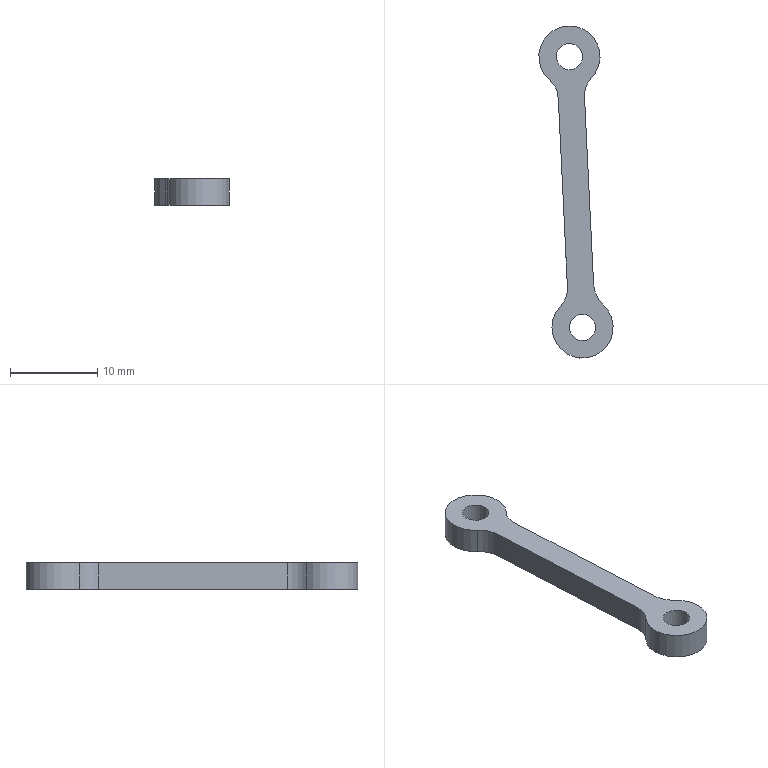Component | NX | LINK_2 | 1 solid | 12 faces | box 8.5 x 37.96 x 3 mm | volume 410 mm3 | cylinder 8 | plane 4 | commonest cylinder face diameters 6 x3 7 x2 3 x2 7.2 x1
STEP:
#1=CARTESIAN_POINT('',(0.,0.,0.));
#2=DIRECTION('',(0.,0.,1.));
#3=DIRECTION('',(1.,0.,0.));
#4=AXIS2_PLACEMENT_3D('',#1,#2,#3);
#5=CARTESIAN_POINT('',(7.782,-30.756,26.65));
#6=VERTEX_POINT('',#5);
#7=CARTESIAN_POINT('',(2.942,-30.99,26.65));
#8=VERTEX_POINT('',#7);
#9=CARTESIAN_POINT('',(5.24,-28.35,26.65));
#10=DIRECTION('',(0.,0.,1.));
#11=DIRECTION('',(0.04829,-0.9988,0.));
#12=AXIS2_PLACEMENT_3D('',#9,#10,#11);
#13=CIRCLE('',#12,3.5);
#14=CARTESIAN_POINT('',(5.24,-28.35,29.65));
#15=DIRECTION('',(0.,0.,-1.));
#16=DIRECTION('',(0.9988,0.04829,0.));
#17=AXIS2_PLACEMENT_3D('',#14,#15,#16);
#18=CYLINDRICAL_SURFACE('',#17,3.5);
#19=CARTESIAN_POINT('',(7.854,3.));
#20=DIRECTION('',(-1.,0.));
#21=VECTOR('',#20,1.);
#22=LINE('',#19,#21);
#23=(GEOMETRIC_REPRESENTATION_CONTEXT(2)PARAMETRIC_REPRESENTATION_CONTEXT()REPRESENTATION_CONTEXT('',''));
#24=DEFINITIONAL_REPRESENTATION('',(#22),#23);
#25=PCURVE('',#18,#24);
#26=CARTESIAN_POINT('',(5.24,-28.35,26.65));
#27=DIRECTION('',(0.,0.,1.));
#28=DIRECTION('',(-0.9988,-0.04829,0.));
#29=AXIS2_PLACEMENT_3D('',#26,#27,#28);
#30=PLANE('',#29);
#31=CARTESIAN_POINT('',(0.,0.));
#32=DIRECTION('',(0.,1.));
#33=AXIS2_PLACEMENT_2D('',#31,#32);
#34=CIRCLE('',#33,3.5);
#35=(GEOMETRIC_REPRESENTATION_CONTEXT(2)PARAMETRIC_REPRESENTATION_CONTEXT()REPRESENTATION_CONTEXT('',''));
#36=DEFINITIONAL_REPRESENTATION('',(#34),#35);
#37=PCURVE('',#30,#36);
#38=SURFACE_CURVE('',#13,(#25,#37),.PCURVE_S1.);
#39=EDGE_CURVE('',#6,#8,#38,.T.);
#40=ORIENTED_EDGE('',*,*,#39,.T.);
#41=CARTESIAN_POINT('',(2.942,-30.99,29.65));
#42=VERTEX_POINT('',#41);
#43=CARTESIAN_POINT('',(2.942,-30.99,29.65));
#44=DIRECTION('',(0.,0.,-1.));
#45=VECTOR('',#44,1.);
#46=LINE('',#43,#45);
#47=CARTESIAN_POINT('',(2.335,0.));
#48=DIRECTION('',(0.,1.));
#49=VECTOR('',#48,1.);
#50=LINE('',#47,#49);
#51=(GEOMETRIC_REPRESENTATION_CONTEXT(2)PARAMETRIC_REPRESENTATION_CONTEXT()REPRESENTATION_CONTEXT('',''));
#52=DEFINITIONAL_REPRESENTATION('',(#50),#51);
#53=PCURVE('',#18,#52);
#54=CARTESIAN_POINT('',(0.9717,-33.252,29.65));
#55=DIRECTION('',(0.,0.,-1.));
#56=DIRECTION('',(0.9988,0.04829,0.));
#57=AXIS2_PLACEMENT_3D('',#54,#55,#56);
#58=CYLINDRICAL_SURFACE('',#57,3.);
#59=CARTESIAN_POINT('',(5.477,0.));
#60=DIRECTION('',(0.,1.));
#61=VECTOR('',#60,1.);
#62=LINE('',#59,#61);
#63=(GEOMETRIC_REPRESENTATION_CONTEXT(2)PARAMETRIC_REPRESENTATION_CONTEXT()REPRESENTATION_CONTEXT('',''));
#64=DEFINITIONAL_REPRESENTATION('',(#62),#63);
#65=PCURVE('',#58,#64);
#66=SURFACE_CURVE('',#46,(#53,#65),.PCURVE_S1.);
#67=EDGE_CURVE('',#42,#8,#66,.T.);
#68=ORIENTED_EDGE('',*,*,#67,.F.);
#69=CARTESIAN_POINT('',(7.782,-30.756,29.65));
#70=VERTEX_POINT('',#69);
#71=CARTESIAN_POINT('',(5.24,-28.35,29.65));
#72=DIRECTION('',(0.,0.,1.));
#73=DIRECTION('',(0.04829,-0.9988,0.));
#74=AXIS2_PLACEMENT_3D('',#71,#72,#73);
#75=CIRCLE('',#74,3.5);
#76=CARTESIAN_POINT('',(7.854,0.));
#77=DIRECTION('',(-1.,0.));
#78=VECTOR('',#77,1.);
#79=LINE('',#76,#78);
#80=(GEOMETRIC_REPRESENTATION_CONTEXT(2)PARAMETRIC_REPRESENTATION_CONTEXT()REPRESENTATION_CONTEXT('',''));
#81=DEFINITIONAL_REPRESENTATION('',(#79),#80);
#82=PCURVE('',#18,#81);
#83=CARTESIAN_POINT('',(5.24,-28.35,29.65));
#84=DIRECTION('',(0.,0.,1.));
#85=DIRECTION('',(-0.9988,-0.04829,0.));
#86=AXIS2_PLACEMENT_3D('',#83,#84,#85);
#87=PLANE('',#86);
#88=CARTESIAN_POINT('',(0.,0.));
#89=DIRECTION('',(0.,1.));
#90=AXIS2_PLACEMENT_2D('',#88,#89);
#91=CIRCLE('',#90,3.5);
#92=(GEOMETRIC_REPRESENTATION_CONTEXT(2)PARAMETRIC_REPRESENTATION_CONTEXT()REPRESENTATION_CONTEXT('',''));
#93=DEFINITIONAL_REPRESENTATION('',(#91),#92);
#94=PCURVE('',#87,#93);
#95=SURFACE_CURVE('',#75,(#82,#94),.PCURVE_S1.);
#96=EDGE_CURVE('',#70,#42,#95,.T.);
#97=ORIENTED_EDGE('',*,*,#96,.F.);
#98=CARTESIAN_POINT('',(7.782,-30.756,29.65));
#99=DIRECTION('',(0.,0.,-1.));
#100=VECTOR('',#99,1.);
#101=LINE('',#98,#100);
#102=CARTESIAN_POINT('',(7.089,0.));
#103=DIRECTION('',(0.,1.));
#104=VECTOR('',#103,1.);
#105=LINE('',#102,#104);
#106=(GEOMETRIC_REPRESENTATION_CONTEXT(2)PARAMETRIC_REPRESENTATION_CONTEXT()REPRESENTATION_CONTEXT('',''));
#107=DEFINITIONAL_REPRESENTATION('',(#105),#106);
#108=PCURVE('',#18,#107);
#109=CARTESIAN_POINT('',(9.961,-32.818,29.65));
#110=DIRECTION('',(0.,0.,-1.));
#111=DIRECTION('',(0.9988,0.04829,0.));
#112=AXIS2_PLACEMENT_3D('',#109,#110,#111);
#113=CYLINDRICAL_SURFACE('',#112,3.);
#114=CARTESIAN_POINT('',(3.948,0.));
#115=DIRECTION('',(0.,1.));
#116=VECTOR('',#115,1.);
#117=LINE('',#114,#116);
#118=(GEOMETRIC_REPRESENTATION_CONTEXT(2)PARAMETRIC_REPRESENTATION_CONTEXT()REPRESENTATION_CONTEXT('',''));
#119=DEFINITIONAL_REPRESENTATION('',(#117),#118);
#120=PCURVE('',#113,#119);
#121=SURFACE_CURVE('',#101,(#108,#120),.PCURVE_S1.);
#122=EDGE_CURVE('',#70,#6,#121,.T.);
#123=ORIENTED_EDGE('',*,*,#122,.T.);
#124=EDGE_LOOP('',(#40,#68,#97,#123));
#125=FACE_BOUND('',#124,.T.);
#126=ADVANCED_FACE('',(#125),#18,.T.);
#127=ORIENTED_EDGE('',*,*,#67,.F.);
#128=CARTESIAN_POINT('',(3.968,-33.107,29.65));
#129=VERTEX_POINT('',#128);
#130=CARTESIAN_POINT('',(0.9717,-33.252,29.65));
#131=DIRECTION('',(0.,0.,-1.));
#132=DIRECTION('',(0.04829,-0.9988,0.));
#133=AXIS2_PLACEMENT_3D('',#130,#131,#132);
#134=CIRCLE('',#133,3.);
#135=CARTESIAN_POINT('',(1.571,0.));
#136=DIRECTION('',(1.,0.));
#137=VECTOR('',#136,1.);
#138=LINE('',#135,#137);
#139=(GEOMETRIC_REPRESENTATION_CONTEXT(2)PARAMETRIC_REPRESENTATION_CONTEXT()REPRESENTATION_CONTEXT('',''));
#140=DEFINITIONAL_REPRESENTATION('',(#138),#139);
#141=PCURVE('',#58,#140);
#142=CARTESIAN_POINT('',(4.5,7.69));
#143=CARTESIAN_POINT('',(9.696,7.69));
#144=CARTESIAN_POINT('',(7.098,3.19));
#145=CARTESIAN_POINT('',(4.5,-1.31));
#146=CARTESIAN_POINT('',(1.902,3.19));
#147=CARTESIAN_POINT('',(-0.6962,7.69));
#148=CARTESIAN_POINT('',(4.5,7.69));
#149=(BOUNDED_CURVE()B_SPLINE_CURVE(2,(#142,#143,#144,#145,#146,#147,#148),.UNSPECIFIED.,.T.,.F.)B_SPLINE_CURVE_WITH_KNOTS((1,2,2,2,2,1),(-2.094,0.,2.094,4.189,6.283,8.378),.UNSPECIFIED.)CURVE()GEOMETRIC_REPRESENTATION_ITEM()RATIONAL_B_SPLINE_CURVE((1.,0.5,1.,0.5,1.,0.5,1.))REPRESENTATION_ITEM(''));
#150=(GEOMETRIC_REPRESENTATION_CONTEXT(2)PARAMETRIC_REPRESENTATION_CONTEXT()REPRESENTATION_CONTEXT('',''));
#151=DEFINITIONAL_REPRESENTATION('',(#149),#150);
#152=PCURVE('',#87,#151);
#153=SURFACE_CURVE('',#134,(#141,#152),.PCURVE_S1.);
#154=EDGE_CURVE('',#42,#129,#153,.T.);
#155=ORIENTED_EDGE('',*,*,#154,.T.);
#156=CARTESIAN_POINT('',(3.968,-33.107,26.65));
#157=VERTEX_POINT('',#156);
#158=CARTESIAN_POINT('',(3.968,-33.107,29.65));
#159=DIRECTION('',(0.,0.,-1.));
#160=VECTOR('',#159,1.);
#161=LINE('',#158,#160);
#162=CARTESIAN_POINT('',(6.283,0.));
#163=DIRECTION('',(0.,1.));
#164=VECTOR('',#163,1.);
#165=LINE('',#162,#164);
#166=(GEOMETRIC_REPRESENTATION_CONTEXT(2)PARAMETRIC_REPRESENTATION_CONTEXT()REPRESENTATION_CONTEXT('',''));
#167=DEFINITIONAL_REPRESENTATION('',(#165),#166);
#168=PCURVE('',#58,#167);
#169=CARTESIAN_POINT('',(3.968,-33.107,29.65));
#170=DIRECTION('',(0.9988,0.04829,0.));
#171=DIRECTION('',(0.04829,-0.9988,0.));
#172=AXIS2_PLACEMENT_3D('',#169,#170,#171);
#173=PLANE('',#172);
#174=CARTESIAN_POINT('',(0.,0.));
#175=DIRECTION('',(0.,1.));
#176=VECTOR('',#175,1.);
#177=LINE('',#174,#176);
#178=(GEOMETRIC_REPRESENTATION_CONTEXT(2)PARAMETRIC_REPRESENTATION_CONTEXT()REPRESENTATION_CONTEXT('',''));
#179=DEFINITIONAL_REPRESENTATION('',(#177),#178);
#180=PCURVE('',#173,#179);
#181=SURFACE_CURVE('',#161,(#168,#180),.PCURVE_S1.);
#182=EDGE_CURVE('',#129,#157,#181,.T.);
#183=ORIENTED_EDGE('',*,*,#182,.T.);
#184=CARTESIAN_POINT('',(0.9717,-33.252,26.65));
#185=DIRECTION('',(0.,0.,-1.));
#186=DIRECTION('',(0.04829,-0.9988,0.));
#187=AXIS2_PLACEMENT_3D('',#184,#185,#186);
#188=CIRCLE('',#187,3.);
#189=CARTESIAN_POINT('',(1.571,3.));
#190=DIRECTION('',(1.,0.));
#191=VECTOR('',#190,1.);
#192=LINE('',#189,#191);
#193=(GEOMETRIC_REPRESENTATION_CONTEXT(2)PARAMETRIC_REPRESENTATION_CONTEXT()REPRESENTATION_CONTEXT('',''));
#194=DEFINITIONAL_REPRESENTATION('',(#192),#193);
#195=PCURVE('',#58,#194);
#196=CARTESIAN_POINT('',(4.5,7.69));
#197=CARTESIAN_POINT('',(9.696,7.69));
#198=CARTESIAN_POINT('',(7.098,3.19));
#199=CARTESIAN_POINT('',(4.5,-1.31));
#200=CARTESIAN_POINT('',(1.902,3.19));
#201=CARTESIAN_POINT('',(-0.6962,7.69));
#202=CARTESIAN_POINT('',(4.5,7.69));
#203=(BOUNDED_CURVE()B_SPLINE_CURVE(2,(#196,#197,#198,#199,#200,#201,#202),.UNSPECIFIED.,.T.,.F.)B_SPLINE_CURVE_WITH_KNOTS((1,2,2,2,2,1),(-2.094,0.,2.094,4.189,6.283,8.378),.UNSPECIFIED.)CURVE()GEOMETRIC_REPRESENTATION_ITEM()RATIONAL_B_SPLINE_CURVE((1.,0.5,1.,0.5,1.,0.5,1.))REPRESENTATION_ITEM(''));
#204=(GEOMETRIC_REPRESENTATION_CONTEXT(2)PARAMETRIC_REPRESENTATION_CONTEXT()REPRESENTATION_CONTEXT('',''));
#205=DEFINITIONAL_REPRESENTATION('',(#203),#204);
#206=PCURVE('',#30,#205);
#207=SURFACE_CURVE('',#188,(#195,#206),.PCURVE_S1.);
#208=EDGE_CURVE('',#8,#157,#207,.T.);
#209=ORIENTED_EDGE('',*,*,#208,.F.);
#210=EDGE_LOOP('',(#127,#155,#183,#209));
#211=FACE_BOUND('',#210,.F.);
#212=ADVANCED_FACE('',(#211),#58,.F.);
#213=CARTESIAN_POINT('',(5.012,-54.701,26.65));
#214=VERTEX_POINT('',#213);
#215=CARTESIAN_POINT('',(3.968,-33.107,26.65));
#216=DIRECTION('',(0.04829,-0.9988,0.));
#217=VECTOR('',#216,1.);
#218=LINE('',#215,#217);
#219=CARTESIAN_POINT('',(0.,3.));
#220=DIRECTION('',(1.,0.));
#221=VECTOR('',#220,1.);
#222=LINE('',#219,#221);
#223=(GEOMETRIC_REPRESENTATION_CONTEXT(2)PARAMETRIC_REPRESENTATION_CONTEXT()REPRESENTATION_CONTEXT('',''));
#224=DEFINITIONAL_REPRESENTATION('',(#222),#223);
#225=PCURVE('',#173,#224);
#226=CARTESIAN_POINT('',(1.5,4.69));
#227=DIRECTION('',(0.,1.));
#228=VECTOR('',#227,1.);
#229=LINE('',#226,#228);
#230=(GEOMETRIC_REPRESENTATION_CONTEXT(2)PARAMETRIC_REPRESENTATION_CONTEXT()REPRESENTATION_CONTEXT('',''));
#231=DEFINITIONAL_REPRESENTATION('',(#229),#230);
#232=PCURVE('',#30,#231);
#233=SURFACE_CURVE('',#218,(#225,#232),.PCURVE_S1.);
#234=EDGE_CURVE('',#157,#214,#233,.T.);
#235=ORIENTED_EDGE('',*,*,#234,.T.);
#236=CARTESIAN_POINT('',(5.012,-54.701,29.65));
#237=VERTEX_POINT('',#236);
#238=CARTESIAN_POINT('',(5.012,-54.701,29.65));
#239=DIRECTION('',(0.,0.,-1.));
#240=VECTOR('',#239,1.);
#241=LINE('',#238,#240);
#242=CARTESIAN_POINT('',(21.619,0.));
#243=DIRECTION('',(0.,1.));
#244=VECTOR('',#243,1.);
#245=LINE('',#242,#244);
#246=(GEOMETRIC_REPRESENTATION_CONTEXT(2)PARAMETRIC_REPRESENTATION_CONTEXT()REPRESENTATION_CONTEXT('',''));
#247=DEFINITIONAL_REPRESENTATION('',(#245),#246);
#248=PCURVE('',#173,#247);
#249=CARTESIAN_POINT('',(2.016,-54.846,29.65));
#250=DIRECTION('',(0.,0.,-1.));
#251=DIRECTION('',(0.9988,0.04829,0.));
#252=AXIS2_PLACEMENT_3D('',#249,#250,#251);
#253=CYLINDRICAL_SURFACE('',#252,3.);
#254=CARTESIAN_POINT('',(0.,0.));
#255=DIRECTION('',(0.,1.));
#256=VECTOR('',#255,1.);
#257=LINE('',#254,#256);
#258=(GEOMETRIC_REPRESENTATION_CONTEXT(2)PARAMETRIC_REPRESENTATION_CONTEXT()REPRESENTATION_CONTEXT('',''));
#259=DEFINITIONAL_REPRESENTATION('',(#257),#258);
#260=PCURVE('',#253,#259);
#261=SURFACE_CURVE('',#241,(#248,#260),.PCURVE_S1.);
#262=EDGE_CURVE('',#237,#214,#261,.T.);
#263=ORIENTED_EDGE('',*,*,#262,.F.);
#264=CARTESIAN_POINT('',(3.968,-33.107,29.65));
#265=DIRECTION('',(0.04829,-0.9988,0.));
#266=VECTOR('',#265,1.);
#267=LINE('',#264,#266);
#268=CARTESIAN_POINT('',(0.,0.));
#269=DIRECTION('',(1.,0.));
#270=VECTOR('',#269,1.);
#271=LINE('',#268,#270);
#272=(GEOMETRIC_REPRESENTATION_CONTEXT(2)PARAMETRIC_REPRESENTATION_CONTEXT()REPRESENTATION_CONTEXT('',''));
#273=DEFINITIONAL_REPRESENTATION('',(#271),#272);
#274=PCURVE('',#173,#273);
#275=CARTESIAN_POINT('',(1.5,4.69));
#276=DIRECTION('',(0.,1.));
#277=VECTOR('',#276,1.);
#278=LINE('',#275,#277);
#279=(GEOMETRIC_REPRESENTATION_CONTEXT(2)PARAMETRIC_REPRESENTATION_CONTEXT()REPRESENTATION_CONTEXT('',''));
#280=DEFINITIONAL_REPRESENTATION('',(#278),#279);
#281=PCURVE('',#87,#280);
#282=SURFACE_CURVE('',#267,(#274,#281),.PCURVE_S1.);
#283=EDGE_CURVE('',#129,#237,#282,.T.);
#284=ORIENTED_EDGE('',*,*,#283,.F.);
#285=ORIENTED_EDGE('',*,*,#182,.T.);
#286=EDGE_LOOP('',(#235,#263,#284,#285));
#287=FACE_BOUND('',#286,.T.);
#288=ADVANCED_FACE('',(#287),#173,.F.);
#289=ORIENTED_EDGE('',*,*,#262,.F.);
#290=CARTESIAN_POINT('',(4.195,-56.908,29.65));
#291=VERTEX_POINT('',#290);
#292=CARTESIAN_POINT('',(2.016,-54.846,29.65));
#293=DIRECTION('',(0.,0.,-1.));
#294=DIRECTION('',(0.04829,-0.9988,0.));
#295=AXIS2_PLACEMENT_3D('',#292,#293,#294);
#296=CIRCLE('',#295,3.);
#297=CARTESIAN_POINT('',(-4.712,0.));
#298=DIRECTION('',(1.,0.));
#299=VECTOR('',#298,1.);
#300=LINE('',#297,#299);
#301=(GEOMETRIC_REPRESENTATION_CONTEXT(2)PARAMETRIC_REPRESENTATION_CONTEXT()REPRESENTATION_CONTEXT('',''));
#302=DEFINITIONAL_REPRESENTATION('',(#300),#301);
#303=PCURVE('',#253,#302);
#304=CARTESIAN_POINT('',(4.5,29.31));
#305=CARTESIAN_POINT('',(9.696,29.31));
#306=CARTESIAN_POINT('',(7.098,24.81));
#307=CARTESIAN_POINT('',(4.5,20.31));
#308=CARTESIAN_POINT('',(1.902,24.81));
#309=CARTESIAN_POINT('',(-0.6962,29.31));
#310=CARTESIAN_POINT('',(4.5,29.31));
#311=(BOUNDED_CURVE()B_SPLINE_CURVE(2,(#304,#305,#306,#307,#308,#309,#310),.UNSPECIFIED.,.T.,.F.)B_SPLINE_CURVE_WITH_KNOTS((1,2,2,2,2,1),(-2.094,0.,2.094,4.189,6.283,8.378),.UNSPECIFIED.)CURVE()GEOMETRIC_REPRESENTATION_ITEM()RATIONAL_B_SPLINE_CURVE((1.,0.5,1.,0.5,1.,0.5,1.))REPRESENTATION_ITEM(''));
#312=(GEOMETRIC_REPRESENTATION_CONTEXT(2)PARAMETRIC_REPRESENTATION_CONTEXT()REPRESENTATION_CONTEXT('',''));
#313=DEFINITIONAL_REPRESENTATION('',(#311),#312);
#314=PCURVE('',#87,#313);
#315=SURFACE_CURVE('',#296,(#303,#314),.PCURVE_S1.);
#316=EDGE_CURVE('',#237,#291,#315,.T.);
#317=ORIENTED_EDGE('',*,*,#316,.T.);
#318=CARTESIAN_POINT('',(4.195,-56.908,26.65));
#319=VERTEX_POINT('',#318);
#320=CARTESIAN_POINT('',(4.195,-56.908,29.65));
#321=DIRECTION('',(0.,0.,-1.));
#322=VECTOR('',#321,1.);
#323=LINE('',#320,#322);
#324=CARTESIAN_POINT('',(0.8061,0.));
#325=DIRECTION('',(0.,1.));
#326=VECTOR('',#325,1.);
#327=LINE('',#324,#326);
#328=(GEOMETRIC_REPRESENTATION_CONTEXT(2)PARAMETRIC_REPRESENTATION_CONTEXT()REPRESENTATION_CONTEXT('',''));
#329=DEFINITIONAL_REPRESENTATION('',(#327),#328);
#330=PCURVE('',#253,#329);
#331=CARTESIAN_POINT('',(6.737,-59.314,29.65));
#332=DIRECTION('',(0.,0.,-1.));
#333=DIRECTION('',(0.9988,0.04829,0.));
#334=AXIS2_PLACEMENT_3D('',#331,#332,#333);
#335=CYLINDRICAL_SURFACE('',#334,3.5);
#336=CARTESIAN_POINT('',(3.948,0.));
#337=DIRECTION('',(0.,1.));
#338=VECTOR('',#337,1.);
#339=LINE('',#336,#338);
#340=(GEOMETRIC_REPRESENTATION_CONTEXT(2)PARAMETRIC_REPRESENTATION_CONTEXT()REPRESENTATION_CONTEXT('',''));
#341=DEFINITIONAL_REPRESENTATION('',(#339),#340);
#342=PCURVE('',#335,#341);
#343=SURFACE_CURVE('',#323,(#330,#342),.PCURVE_S1.);
#344=EDGE_CURVE('',#291,#319,#343,.T.);
#345=ORIENTED_EDGE('',*,*,#344,.T.);
#346=CARTESIAN_POINT('',(2.016,-54.846,26.65));
#347=DIRECTION('',(0.,0.,-1.));
#348=DIRECTION('',(0.04829,-0.9988,0.));
#349=AXIS2_PLACEMENT_3D('',#346,#347,#348);
#350=CIRCLE('',#349,3.);
#351=CARTESIAN_POINT('',(-4.712,3.));
#352=DIRECTION('',(1.,0.));
#353=VECTOR('',#352,1.);
#354=LINE('',#351,#353);
#355=(GEOMETRIC_REPRESENTATION_CONTEXT(2)PARAMETRIC_REPRESENTATION_CONTEXT()REPRESENTATION_CONTEXT('',''));
#356=DEFINITIONAL_REPRESENTATION('',(#354),#355);
#357=PCURVE('',#253,#356);
#358=CARTESIAN_POINT('',(4.5,29.31));
#359=CARTESIAN_POINT('',(9.696,29.31));
#360=CARTESIAN_POINT('',(7.098,24.81));
#361=CARTESIAN_POINT('',(4.5,20.31));
#362=CARTESIAN_POINT('',(1.902,24.81));
#363=CARTESIAN_POINT('',(-0.6962,29.31));
#364=CARTESIAN_POINT('',(4.5,29.31));
#365=(BOUNDED_CURVE()B_SPLINE_CURVE(2,(#358,#359,#360,#361,#362,#363,#364),.UNSPECIFIED.,.T.,.F.)B_SPLINE_CURVE_WITH_KNOTS((1,2,2,2,2,1),(-2.094,0.,2.094,4.189,6.283,8.378),.UNSPECIFIED.)CURVE()GEOMETRIC_REPRESENTATION_ITEM()RATIONAL_B_SPLINE_CURVE((1.,0.5,1.,0.5,1.,0.5,1.))REPRESENTATION_ITEM(''));
#366=(GEOMETRIC_REPRESENTATION_CONTEXT(2)PARAMETRIC_REPRESENTATION_CONTEXT()REPRESENTATION_CONTEXT('',''));
#367=DEFINITIONAL_REPRESENTATION('',(#365),#366);
#368=PCURVE('',#30,#367);
#369=SURFACE_CURVE('',#350,(#357,#368),.PCURVE_S1.);
#370=EDGE_CURVE('',#214,#319,#369,.T.);
#371=ORIENTED_EDGE('',*,*,#370,.F.);
#372=EDGE_LOOP('',(#289,#317,#345,#371));
#373=FACE_BOUND('',#372,.F.);
#374=ADVANCED_FACE('',(#373),#253,.F.);
#375=CARTESIAN_POINT('',(9.13,-56.76,26.65));
#376=VERTEX_POINT('',#375);
#377=CARTESIAN_POINT('',(6.737,-59.314,26.65));
#378=DIRECTION('',(0.,0.,1.));
#379=DIRECTION('',(0.04829,-0.9988,0.));
#380=AXIS2_PLACEMENT_3D('',#377,#378,#379);
#381=CIRCLE('',#380,3.5);
#382=CARTESIAN_POINT('',(7.854,3.));
#383=DIRECTION('',(-1.,0.));
#384=VECTOR('',#383,1.);
#385=LINE('',#382,#384);
#386=(GEOMETRIC_REPRESENTATION_CONTEXT(2)PARAMETRIC_REPRESENTATION_CONTEXT()REPRESENTATION_CONTEXT('',''));
#387=DEFINITIONAL_REPRESENTATION('',(#385),#386);
#388=PCURVE('',#335,#387);
#389=CARTESIAN_POINT('',(0.,31.));
#390=DIRECTION('',(0.,1.));
#391=AXIS2_PLACEMENT_2D('',#389,#390);
#392=CIRCLE('',#391,3.5);
#393=(GEOMETRIC_REPRESENTATION_CONTEXT(2)PARAMETRIC_REPRESENTATION_CONTEXT()REPRESENTATION_CONTEXT('',''));
#394=DEFINITIONAL_REPRESENTATION('',(#392),#393);
#395=PCURVE('',#30,#394);
#396=SURFACE_CURVE('',#381,(#388,#395),.PCURVE_S1.);
#397=EDGE_CURVE('',#319,#376,#396,.T.);
#398=ORIENTED_EDGE('',*,*,#397,.T.);
#399=CARTESIAN_POINT('',(9.13,-56.76,29.65));
#400=VERTEX_POINT('',#399);
#401=CARTESIAN_POINT('',(9.13,-56.76,29.65));
#402=DIRECTION('',(0.,0.,-1.));
#403=VECTOR('',#402,1.);
#404=LINE('',#401,#403);
#405=CARTESIAN_POINT('',(-0.7694,0.));
#406=DIRECTION('',(0.,1.));
#407=VECTOR('',#406,1.);
#408=LINE('',#405,#407);
#409=(GEOMETRIC_REPRESENTATION_CONTEXT(2)PARAMETRIC_REPRESENTATION_CONTEXT()REPRESENTATION_CONTEXT('',''));
#410=DEFINITIONAL_REPRESENTATION('',(#408),#409);
#411=PCURVE('',#335,#410);
#412=CARTESIAN_POINT('',(11.592,-54.134,29.65));
#413=DIRECTION('',(0.,0.,-1.));
#414=DIRECTION('',(0.9988,0.04829,0.));
#415=AXIS2_PLACEMENT_3D('',#412,#413,#414);
#416=CYLINDRICAL_SURFACE('',#415,3.6);
#417=CARTESIAN_POINT('',(2.372,0.));
#418=DIRECTION('',(0.,1.));
#419=VECTOR('',#418,1.);
#420=LINE('',#417,#419);
#421=(GEOMETRIC_REPRESENTATION_CONTEXT(2)PARAMETRIC_REPRESENTATION_CONTEXT()REPRESENTATION_CONTEXT('',''));
#422=DEFINITIONAL_REPRESENTATION('',(#420),#421);
#423=PCURVE('',#416,#422);
#424=SURFACE_CURVE('',#404,(#411,#423),.PCURVE_S1.);
#425=EDGE_CURVE('',#400,#376,#424,.T.);
#426=ORIENTED_EDGE('',*,*,#425,.F.);
#427=CARTESIAN_POINT('',(6.737,-59.314,29.65));
#428=DIRECTION('',(0.,0.,1.));
#429=DIRECTION('',(0.04829,-0.9988,0.));
#430=AXIS2_PLACEMENT_3D('',#427,#428,#429);
#431=CIRCLE('',#430,3.5);
#432=CARTESIAN_POINT('',(7.854,0.));
#433=DIRECTION('',(-1.,0.));
#434=VECTOR('',#433,1.);
#435=LINE('',#432,#434);
#436=(GEOMETRIC_REPRESENTATION_CONTEXT(2)PARAMETRIC_REPRESENTATION_CONTEXT()REPRESENTATION_CONTEXT('',''));
#437=DEFINITIONAL_REPRESENTATION('',(#435),#436);
#438=PCURVE('',#335,#437);
#439=CARTESIAN_POINT('',(0.,31.));
#440=DIRECTION('',(0.,1.));
#441=AXIS2_PLACEMENT_2D('',#439,#440);
#442=CIRCLE('',#441,3.5);
#443=(GEOMETRIC_REPRESENTATION_CONTEXT(2)PARAMETRIC_REPRESENTATION_CONTEXT()REPRESENTATION_CONTEXT('',''));
#444=DEFINITIONAL_REPRESENTATION('',(#442),#443);
#445=PCURVE('',#87,#444);
#446=SURFACE_CURVE('',#431,(#438,#445),.PCURVE_S1.);
#447=EDGE_CURVE('',#291,#400,#446,.T.);
#448=ORIENTED_EDGE('',*,*,#447,.F.);
#449=ORIENTED_EDGE('',*,*,#344,.T.);
#450=EDGE_LOOP('',(#398,#426,#448,#449));
#451=FACE_BOUND('',#450,.T.);
#452=ADVANCED_FACE('',(#451),#335,.T.);
#453=ORIENTED_EDGE('',*,*,#425,.F.);
#454=CARTESIAN_POINT('',(7.997,-54.308,29.65));
#455=VERTEX_POINT('',#454);
#456=CARTESIAN_POINT('',(11.592,-54.134,29.65));
#457=DIRECTION('',(0.,0.,-1.));
#458=DIRECTION('',(0.04829,-0.9988,0.));
#459=AXIS2_PLACEMENT_3D('',#456,#457,#458);
#460=CIRCLE('',#459,3.6);
#461=CARTESIAN_POINT('',(1.571,0.));
#462=DIRECTION('',(1.,0.));
#463=VECTOR('',#462,1.);
#464=LINE('',#461,#463);
#465=(GEOMETRIC_REPRESENTATION_CONTEXT(2)PARAMETRIC_REPRESENTATION_CONTEXT()REPRESENTATION_CONTEXT('',''));
#466=DEFINITIONAL_REPRESENTATION('',(#464),#465);
#467=PCURVE('',#416,#466);
#468=CARTESIAN_POINT('',(-5.1,29.66));
#469=CARTESIAN_POINT('',(1.135,29.66));
#470=CARTESIAN_POINT('',(-1.982,24.26));
#471=CARTESIAN_POINT('',(-5.1,18.86));
#472=CARTESIAN_POINT('',(-8.218,24.26));
#473=CARTESIAN_POINT('',(-11.335,29.66));
#474=CARTESIAN_POINT('',(-5.1,29.66));
#475=(BOUNDED_CURVE()B_SPLINE_CURVE(2,(#468,#469,#470,#471,#472,#473,#474),.UNSPECIFIED.,.T.,.F.)B_SPLINE_CURVE_WITH_KNOTS((1,2,2,2,2,1),(-2.094,0.,2.094,4.189,6.283,8.378),.UNSPECIFIED.)CURVE()GEOMETRIC_REPRESENTATION_ITEM()RATIONAL_B_SPLINE_CURVE((1.,0.5,1.,0.5,1.,0.5,1.))REPRESENTATION_ITEM(''));
#476=(GEOMETRIC_REPRESENTATION_CONTEXT(2)PARAMETRIC_REPRESENTATION_CONTEXT()REPRESENTATION_CONTEXT('',''));
#477=DEFINITIONAL_REPRESENTATION('',(#475),#476);
#478=PCURVE('',#87,#477);
#479=SURFACE_CURVE('',#460,(#467,#478),.PCURVE_S1.);
#480=EDGE_CURVE('',#400,#455,#479,.T.);
#481=ORIENTED_EDGE('',*,*,#480,.T.);
#482=CARTESIAN_POINT('',(7.997,-54.308,26.65));
#483=VERTEX_POINT('',#482);
#484=CARTESIAN_POINT('',(7.997,-54.308,29.65));
#485=DIRECTION('',(0.,0.,-1.));
#486=VECTOR('',#485,1.);
#487=LINE('',#484,#486);
#488=CARTESIAN_POINT('',(3.142,0.));
#489=DIRECTION('',(0.,1.));
#490=VECTOR('',#489,1.);
#491=LINE('',#488,#490);
#492=(GEOMETRIC_REPRESENTATION_CONTEXT(2)PARAMETRIC_REPRESENTATION_CONTEXT()REPRESENTATION_CONTEXT('',''));
#493=DEFINITIONAL_REPRESENTATION('',(#491),#492);
#494=PCURVE('',#416,#493);
#495=CARTESIAN_POINT('',(7.997,-54.308,29.65));
#496=DIRECTION('',(-0.9988,-0.04829,0.));
#497=DIRECTION('',(-0.04829,0.9988,0.));
#498=AXIS2_PLACEMENT_3D('',#495,#496,#497);
#499=PLANE('',#498);
#500=CARTESIAN_POINT('',(0.,0.));
#501=DIRECTION('',(0.,1.));
#502=VECTOR('',#501,1.);
#503=LINE('',#500,#502);
#504=(GEOMETRIC_REPRESENTATION_CONTEXT(2)PARAMETRIC_REPRESENTATION_CONTEXT()REPRESENTATION_CONTEXT('',''));
#505=DEFINITIONAL_REPRESENTATION('',(#503),#504);
#506=PCURVE('',#499,#505);
#507=SURFACE_CURVE('',#487,(#494,#506),.PCURVE_S1.);
#508=EDGE_CURVE('',#455,#483,#507,.T.);
#509=ORIENTED_EDGE('',*,*,#508,.T.);
#510=CARTESIAN_POINT('',(11.592,-54.134,26.65));
#511=DIRECTION('',(0.,0.,-1.));
#512=DIRECTION('',(0.04829,-0.9988,0.));
#513=AXIS2_PLACEMENT_3D('',#510,#511,#512);
#514=CIRCLE('',#513,3.6);
#515=CARTESIAN_POINT('',(1.571,3.));
#516=DIRECTION('',(1.,0.));
#517=VECTOR('',#516,1.);
#518=LINE('',#515,#517);
#519=(GEOMETRIC_REPRESENTATION_CONTEXT(2)PARAMETRIC_REPRESENTATION_CONTEXT()REPRESENTATION_CONTEXT('',''));
#520=DEFINITIONAL_REPRESENTATION('',(#518),#519);
#521=PCURVE('',#416,#520);
#522=CARTESIAN_POINT('',(-5.1,29.66));
#523=CARTESIAN_POINT('',(1.135,29.66));
#524=CARTESIAN_POINT('',(-1.982,24.26));
#525=CARTESIAN_POINT('',(-5.1,18.86));
#526=CARTESIAN_POINT('',(-8.218,24.26));
#527=CARTESIAN_POINT('',(-11.335,29.66));
#528=CARTESIAN_POINT('',(-5.1,29.66));
#529=(BOUNDED_CURVE()B_SPLINE_CURVE(2,(#522,#523,#524,#525,#526,#527,#528),.UNSPECIFIED.,.T.,.F.)B_SPLINE_CURVE_WITH_KNOTS((1,2,2,2,2,1),(-2.094,0.,2.094,4.189,6.283,8.378),.UNSPECIFIED.)CURVE()GEOMETRIC_REPRESENTATION_ITEM()RATIONAL_B_SPLINE_CURVE((1.,0.5,1.,0.5,1.,0.5,1.))REPRESENTATION_ITEM(''));
#530=(GEOMETRIC_REPRESENTATION_CONTEXT(2)PARAMETRIC_REPRESENTATION_CONTEXT()REPRESENTATION_CONTEXT('',''));
#531=DEFINITIONAL_REPRESENTATION('',(#529),#530);
#532=PCURVE('',#30,#531);
#533=SURFACE_CURVE('',#514,(#521,#532),.PCURVE_S1.);
#534=EDGE_CURVE('',#376,#483,#533,.T.);
#535=ORIENTED_EDGE('',*,*,#534,.F.);
#536=EDGE_LOOP('',(#453,#481,#509,#535));
#537=FACE_BOUND('',#536,.F.);
#538=ADVANCED_FACE('',(#537),#416,.F.);
#539=CARTESIAN_POINT('',(6.965,-32.963,26.65));
#540=VERTEX_POINT('',#539);
#541=CARTESIAN_POINT('',(7.997,-54.308,26.65));
#542=DIRECTION('',(-0.04829,0.9988,0.));
#543=VECTOR('',#542,1.);
#544=LINE('',#541,#543);
#545=CARTESIAN_POINT('',(0.,3.));
#546=DIRECTION('',(1.,0.));
#547=VECTOR('',#546,1.);
#548=LINE('',#545,#547);
#549=(GEOMETRIC_REPRESENTATION_CONTEXT(2)PARAMETRIC_REPRESENTATION_CONTEXT()REPRESENTATION_CONTEXT('',''));
#550=DEFINITIONAL_REPRESENTATION('',(#548),#549);
#551=PCURVE('',#499,#550);
#552=CARTESIAN_POINT('',(-1.5,26.06));
#553=DIRECTION('',(0.,-1.));
#554=VECTOR('',#553,1.);
#555=LINE('',#552,#554);
#556=(GEOMETRIC_REPRESENTATION_CONTEXT(2)PARAMETRIC_REPRESENTATION_CONTEXT()REPRESENTATION_CONTEXT('',''));
#557=DEFINITIONAL_REPRESENTATION('',(#555),#556);
#558=PCURVE('',#30,#557);
#559=SURFACE_CURVE('',#544,(#551,#558),.PCURVE_S1.);
#560=EDGE_CURVE('',#483,#540,#559,.T.);
#561=ORIENTED_EDGE('',*,*,#560,.T.);
#562=CARTESIAN_POINT('',(6.965,-32.963,29.65));
#563=VERTEX_POINT('',#562);
#564=CARTESIAN_POINT('',(6.965,-32.963,29.65));
#565=DIRECTION('',(0.,0.,-1.));
#566=VECTOR('',#565,1.);
#567=LINE('',#564,#566);
#568=CARTESIAN_POINT('',(21.37,0.));
#569=DIRECTION('',(0.,1.));
#570=VECTOR('',#569,1.);
#571=LINE('',#568,#570);
#572=(GEOMETRIC_REPRESENTATION_CONTEXT(2)PARAMETRIC_REPRESENTATION_CONTEXT()REPRESENTATION_CONTEXT('',''));
#573=DEFINITIONAL_REPRESENTATION('',(#571),#572);
#574=PCURVE('',#499,#573);
#575=CARTESIAN_POINT('',(3.142,0.));
#576=DIRECTION('',(0.,1.));
#577=VECTOR('',#576,1.);
#578=LINE('',#575,#577);
#579=(GEOMETRIC_REPRESENTATION_CONTEXT(2)PARAMETRIC_REPRESENTATION_CONTEXT()REPRESENTATION_CONTEXT('',''));
#580=DEFINITIONAL_REPRESENTATION('',(#578),#579);
#581=PCURVE('',#113,#580);
#582=SURFACE_CURVE('',#567,(#574,#581),.PCURVE_S1.);
#583=EDGE_CURVE('',#563,#540,#582,.T.);
#584=ORIENTED_EDGE('',*,*,#583,.F.);
#585=CARTESIAN_POINT('',(7.997,-54.308,29.65));
#586=DIRECTION('',(-0.04829,0.9988,0.));
#587=VECTOR('',#586,1.);
#588=LINE('',#585,#587);
#589=CARTESIAN_POINT('',(0.,0.));
#590=DIRECTION('',(1.,0.));
#591=VECTOR('',#590,1.);
#592=LINE('',#589,#591);
#593=(GEOMETRIC_REPRESENTATION_CONTEXT(2)PARAMETRIC_REPRESENTATION_CONTEXT()REPRESENTATION_CONTEXT('',''));
#594=DEFINITIONAL_REPRESENTATION('',(#592),#593);
#595=PCURVE('',#499,#594);
#596=CARTESIAN_POINT('',(-1.5,26.06));
#597=DIRECTION('',(0.,-1.));
#598=VECTOR('',#597,1.);
#599=LINE('',#596,#598);
#600=(GEOMETRIC_REPRESENTATION_CONTEXT(2)PARAMETRIC_REPRESENTATION_CONTEXT()REPRESENTATION_CONTEXT('',''));
#601=DEFINITIONAL_REPRESENTATION('',(#599),#600);
#602=PCURVE('',#87,#601);
#603=SURFACE_CURVE('',#588,(#595,#602),.PCURVE_S1.);
#604=EDGE_CURVE('',#455,#563,#603,.T.);
#605=ORIENTED_EDGE('',*,*,#604,.F.);
#606=ORIENTED_EDGE('',*,*,#508,.T.);
#607=EDGE_LOOP('',(#561,#584,#605,#606));
#608=FACE_BOUND('',#607,.T.);
#609=ADVANCED_FACE('',(#608),#499,.F.);
#610=CARTESIAN_POINT('',(5.312,-29.848,29.65));
#611=VERTEX_POINT('',#610);
#612=CARTESIAN_POINT('',(5.24,-28.35,29.65));
#613=DIRECTION('',(0.,0.,1.));
#614=DIRECTION('',(0.04829,-0.9988,0.));
#615=AXIS2_PLACEMENT_3D('',#612,#613,#614);
#616=CIRCLE('',#615,1.5);
#617=CARTESIAN_POINT('',(5.24,-28.35,29.65));
#618=DIRECTION('',(0.,0.,-1.));
#619=DIRECTION('',(0.9988,0.04829,0.));
#620=AXIS2_PLACEMENT_3D('',#617,#618,#619);
#621=CYLINDRICAL_SURFACE('',#620,1.5);
#622=CARTESIAN_POINT('',(7.854,0.));
#623=DIRECTION('',(-1.,0.));
#624=VECTOR('',#623,1.);
#625=LINE('',#622,#624);
#626=(GEOMETRIC_REPRESENTATION_CONTEXT(2)PARAMETRIC_REPRESENTATION_CONTEXT()REPRESENTATION_CONTEXT('',''));
#627=DEFINITIONAL_REPRESENTATION('',(#625),#626);
#628=PCURVE('',#621,#627);
#629=CARTESIAN_POINT('',(0.,0.));
#630=DIRECTION('',(0.,1.));
#631=AXIS2_PLACEMENT_2D('',#629,#630);
#632=CIRCLE('',#631,1.5);
#633=(GEOMETRIC_REPRESENTATION_CONTEXT(2)PARAMETRIC_REPRESENTATION_CONTEXT()REPRESENTATION_CONTEXT('',''));
#634=DEFINITIONAL_REPRESENTATION('',(#632),#633);
#635=PCURVE('',#87,#634);
#636=SURFACE_CURVE('',#616,(#628,#635),.PCURVE_S1.);
#637=EDGE_CURVE('',#611,#611,#636,.T.);
#638=ORIENTED_EDGE('',*,*,#637,.F.);
#639=CARTESIAN_POINT('',(5.312,-29.848,26.65));
#640=VERTEX_POINT('',#639);
#641=CARTESIAN_POINT('',(5.312,-29.848,29.65));
#642=CARTESIAN_POINT('',(5.312,-29.848,26.65));
#643=B_SPLINE_CURVE_WITH_KNOTS('',1,(#641,#642),.UNSPECIFIED.,.F.,.F.,(2,2),(0.,3.),.PIECEWISE_BEZIER_KNOTS.);
#644=CARTESIAN_POINT('',(7.854,0.));
#645=DIRECTION('',(0.,1.));
#646=VECTOR('',#645,1.);
#647=LINE('',#644,#646);
#648=(GEOMETRIC_REPRESENTATION_CONTEXT(2)PARAMETRIC_REPRESENTATION_CONTEXT()REPRESENTATION_CONTEXT('',''));
#649=DEFINITIONAL_REPRESENTATION('',(#647),#648);
#650=PCURVE('',#621,#649);
#651=CARTESIAN_POINT('',(1.571,0.));
#652=DIRECTION('',(0.,1.));
#653=VECTOR('',#652,1.);
#654=LINE('',#651,#653);
#655=(GEOMETRIC_REPRESENTATION_CONTEXT(2)PARAMETRIC_REPRESENTATION_CONTEXT()REPRESENTATION_CONTEXT('',''));
#656=DEFINITIONAL_REPRESENTATION('',(#654),#655);
#657=PCURVE('',#621,#656);
#658=SEAM_CURVE('',#643,(#650,#657),.PCURVE_S1.);
#659=EDGE_CURVE('',#611,#640,#658,.T.);
#660=ORIENTED_EDGE('',*,*,#659,.T.);
#661=CARTESIAN_POINT('',(5.24,-28.35,26.65));
#662=DIRECTION('',(0.,0.,1.));
#663=DIRECTION('',(0.04829,-0.9988,0.));
#664=AXIS2_PLACEMENT_3D('',#661,#662,#663);
#665=CIRCLE('',#664,1.5);
#666=CARTESIAN_POINT('',(7.854,3.));
#667=DIRECTION('',(-1.,0.));
#668=VECTOR('',#667,1.);
#669=LINE('',#666,#668);
#670=(GEOMETRIC_REPRESENTATION_CONTEXT(2)PARAMETRIC_REPRESENTATION_CONTEXT()REPRESENTATION_CONTEXT('',''));
#671=DEFINITIONAL_REPRESENTATION('',(#669),#670);
#672=PCURVE('',#621,#671);
#673=CARTESIAN_POINT('',(0.,0.));
#674=DIRECTION('',(0.,1.));
#675=AXIS2_PLACEMENT_2D('',#673,#674);
#676=CIRCLE('',#675,1.5);
#677=(GEOMETRIC_REPRESENTATION_CONTEXT(2)PARAMETRIC_REPRESENTATION_CONTEXT()REPRESENTATION_CONTEXT('',''));
#678=DEFINITIONAL_REPRESENTATION('',(#676),#677);
#679=PCURVE('',#30,#678);
#680=SURFACE_CURVE('',#665,(#672,#679),.PCURVE_S1.);
#681=EDGE_CURVE('',#640,#640,#680,.T.);
#682=ORIENTED_EDGE('',*,*,#681,.T.);
#683=ORIENTED_EDGE('',*,*,#659,.F.);
#684=EDGE_LOOP('',(#638,#660,#682,#683));
#685=FACE_BOUND('',#684,.F.);
#686=ADVANCED_FACE('',(#685),#621,.F.);
#687=ORIENTED_EDGE('',*,*,#583,.F.);
#688=CARTESIAN_POINT('',(9.961,-32.818,29.65));
#689=DIRECTION('',(0.,0.,-1.));
#690=DIRECTION('',(0.04829,-0.9988,0.));
#691=AXIS2_PLACEMENT_3D('',#688,#689,#690);
#692=CIRCLE('',#691,3.);
#693=CARTESIAN_POINT('',(1.571,0.));
#694=DIRECTION('',(1.,0.));
#695=VECTOR('',#694,1.);
#696=LINE('',#693,#695);
#697=(GEOMETRIC_REPRESENTATION_CONTEXT(2)PARAMETRIC_REPRESENTATION_CONTEXT()REPRESENTATION_CONTEXT('',''));
#698=DEFINITIONAL_REPRESENTATION('',(#696),#697);
#699=PCURVE('',#113,#698);
#700=CARTESIAN_POINT('',(-4.5,7.69));
#701=CARTESIAN_POINT('',(0.6962,7.69));
#702=CARTESIAN_POINT('',(-1.902,3.19));
#703=CARTESIAN_POINT('',(-4.5,-1.31));
#704=CARTESIAN_POINT('',(-7.098,3.19));
#705=CARTESIAN_POINT('',(-9.696,7.69));
#706=CARTESIAN_POINT('',(-4.5,7.69));
#707=(BOUNDED_CURVE()B_SPLINE_CURVE(2,(#700,#701,#702,#703,#704,#705,#706),.UNSPECIFIED.,.T.,.F.)B_SPLINE_CURVE_WITH_KNOTS((1,2,2,2,2,1),(-2.094,0.,2.094,4.189,6.283,8.378),.UNSPECIFIED.)CURVE()GEOMETRIC_REPRESENTATION_ITEM()RATIONAL_B_SPLINE_CURVE((1.,0.5,1.,0.5,1.,0.5,1.))REPRESENTATION_ITEM(''));
#708=(GEOMETRIC_REPRESENTATION_CONTEXT(2)PARAMETRIC_REPRESENTATION_CONTEXT()REPRESENTATION_CONTEXT('',''));
#709=DEFINITIONAL_REPRESENTATION('',(#707),#708);
#710=PCURVE('',#87,#709);
#711=SURFACE_CURVE('',#692,(#699,#710),.PCURVE_S1.);
#712=EDGE_CURVE('',#563,#70,#711,.T.);
#713=ORIENTED_EDGE('',*,*,#712,.T.);
#714=ORIENTED_EDGE('',*,*,#122,.T.);
#715=CARTESIAN_POINT('',(9.961,-32.818,26.65));
#716=DIRECTION('',(0.,0.,-1.));
#717=DIRECTION('',(0.04829,-0.9988,0.));
#718=AXIS2_PLACEMENT_3D('',#715,#716,#717);
#719=CIRCLE('',#718,3.);
#720=CARTESIAN_POINT('',(1.571,3.));
#721=DIRECTION('',(1.,0.));
#722=VECTOR('',#721,1.);
#723=LINE('',#720,#722);
#724=(GEOMETRIC_REPRESENTATION_CONTEXT(2)PARAMETRIC_REPRESENTATION_CONTEXT()REPRESENTATION_CONTEXT('',''));
#725=DEFINITIONAL_REPRESENTATION('',(#723),#724);
#726=PCURVE('',#113,#725);
#727=CARTESIAN_POINT('',(-4.5,7.69));
#728=CARTESIAN_POINT('',(0.6962,7.69));
#729=CARTESIAN_POINT('',(-1.902,3.19));
#730=CARTESIAN_POINT('',(-4.5,-1.31));
#731=CARTESIAN_POINT('',(-7.098,3.19));
#732=CARTESIAN_POINT('',(-9.696,7.69));
#733=CARTESIAN_POINT('',(-4.5,7.69));
#734=(BOUNDED_CURVE()B_SPLINE_CURVE(2,(#727,#728,#729,#730,#731,#732,#733),.UNSPECIFIED.,.T.,.F.)B_SPLINE_CURVE_WITH_KNOTS((1,2,2,2,2,1),(-2.094,0.,2.094,4.189,6.283,8.378),.UNSPECIFIED.)CURVE()GEOMETRIC_REPRESENTATION_ITEM()RATIONAL_B_SPLINE_CURVE((1.,0.5,1.,0.5,1.,0.5,1.))REPRESENTATION_ITEM(''));
#735=(GEOMETRIC_REPRESENTATION_CONTEXT(2)PARAMETRIC_REPRESENTATION_CONTEXT()REPRESENTATION_CONTEXT('',''));
#736=DEFINITIONAL_REPRESENTATION('',(#734),#735);
#737=PCURVE('',#30,#736);
#738=SURFACE_CURVE('',#719,(#726,#737),.PCURVE_S1.);
#739=EDGE_CURVE('',#540,#6,#738,.T.);
#740=ORIENTED_EDGE('',*,*,#739,.F.);
#741=EDGE_LOOP('',(#687,#713,#714,#740));
#742=FACE_BOUND('',#741,.F.);
#743=ADVANCED_FACE('',(#742),#113,.F.);
#744=CARTESIAN_POINT('',(6.809,-60.812,29.65));
#745=VERTEX_POINT('',#744);
#746=CARTESIAN_POINT('',(6.737,-59.314,29.65));
#747=DIRECTION('',(0.,0.,1.));
#748=DIRECTION('',(0.04829,-0.9988,0.));
#749=AXIS2_PLACEMENT_3D('',#746,#747,#748);
#750=CIRCLE('',#749,1.5);
#751=CARTESIAN_POINT('',(6.737,-59.314,29.65));
#752=DIRECTION('',(0.,0.,-1.));
#753=DIRECTION('',(0.9988,0.04829,0.));
#754=AXIS2_PLACEMENT_3D('',#751,#752,#753);
#755=CYLINDRICAL_SURFACE('',#754,1.5);
#756=CARTESIAN_POINT('',(7.854,0.));
#757=DIRECTION('',(-1.,0.));
#758=VECTOR('',#757,1.);
#759=LINE('',#756,#758);
#760=(GEOMETRIC_REPRESENTATION_CONTEXT(2)PARAMETRIC_REPRESENTATION_CONTEXT()REPRESENTATION_CONTEXT('',''));
#761=DEFINITIONAL_REPRESENTATION('',(#759),#760);
#762=PCURVE('',#755,#761);
#763=CARTESIAN_POINT('',(0.,31.));
#764=DIRECTION('',(0.,1.));
#765=AXIS2_PLACEMENT_2D('',#763,#764);
#766=CIRCLE('',#765,1.5);
#767=(GEOMETRIC_REPRESENTATION_CONTEXT(2)PARAMETRIC_REPRESENTATION_CONTEXT()REPRESENTATION_CONTEXT('',''));
#768=DEFINITIONAL_REPRESENTATION('',(#766),#767);
#769=PCURVE('',#87,#768);
#770=SURFACE_CURVE('',#750,(#762,#769),.PCURVE_S1.);
#771=EDGE_CURVE('',#745,#745,#770,.T.);
#772=ORIENTED_EDGE('',*,*,#771,.F.);
#773=CARTESIAN_POINT('',(6.809,-60.812,26.65));
#774=VERTEX_POINT('',#773);
#775=CARTESIAN_POINT('',(6.809,-60.812,29.65));
#776=CARTESIAN_POINT('',(6.809,-60.812,26.65));
#777=B_SPLINE_CURVE_WITH_KNOTS('',1,(#775,#776),.UNSPECIFIED.,.F.,.F.,(2,2),(0.,3.),.PIECEWISE_BEZIER_KNOTS.);
#778=CARTESIAN_POINT('',(7.854,0.));
#779=DIRECTION('',(0.,1.));
#780=VECTOR('',#779,1.);
#781=LINE('',#778,#780);
#782=(GEOMETRIC_REPRESENTATION_CONTEXT(2)PARAMETRIC_REPRESENTATION_CONTEXT()REPRESENTATION_CONTEXT('',''));
#783=DEFINITIONAL_REPRESENTATION('',(#781),#782);
#784=PCURVE('',#755,#783);
#785=CARTESIAN_POINT('',(1.571,0.));
#786=DIRECTION('',(0.,1.));
#787=VECTOR('',#786,1.);
#788=LINE('',#785,#787);
#789=(GEOMETRIC_REPRESENTATION_CONTEXT(2)PARAMETRIC_REPRESENTATION_CONTEXT()REPRESENTATION_CONTEXT('',''));
#790=DEFINITIONAL_REPRESENTATION('',(#788),#789);
#791=PCURVE('',#755,#790);
#792=SEAM_CURVE('',#777,(#784,#791),.PCURVE_S1.);
#793=EDGE_CURVE('',#745,#774,#792,.T.);
#794=ORIENTED_EDGE('',*,*,#793,.T.);
#795=CARTESIAN_POINT('',(6.737,-59.314,26.65));
#796=DIRECTION('',(0.,0.,1.));
#797=DIRECTION('',(0.04829,-0.9988,0.));
#798=AXIS2_PLACEMENT_3D('',#795,#796,#797);
#799=CIRCLE('',#798,1.5);
#800=CARTESIAN_POINT('',(7.854,3.));
#801=DIRECTION('',(-1.,0.));
#802=VECTOR('',#801,1.);
#803=LINE('',#800,#802);
#804=(GEOMETRIC_REPRESENTATION_CONTEXT(2)PARAMETRIC_REPRESENTATION_CONTEXT()REPRESENTATION_CONTEXT('',''));
#805=DEFINITIONAL_REPRESENTATION('',(#803),#804);
#806=PCURVE('',#755,#805);
#807=CARTESIAN_POINT('',(0.,31.));
#808=DIRECTION('',(0.,1.));
#809=AXIS2_PLACEMENT_2D('',#807,#808);
#810=CIRCLE('',#809,1.5);
#811=(GEOMETRIC_REPRESENTATION_CONTEXT(2)PARAMETRIC_REPRESENTATION_CONTEXT()REPRESENTATION_CONTEXT('',''));
#812=DEFINITIONAL_REPRESENTATION('',(#810),#811);
#813=PCURVE('',#30,#812);
#814=SURFACE_CURVE('',#799,(#806,#813),.PCURVE_S1.);
#815=EDGE_CURVE('',#774,#774,#814,.T.);
#816=ORIENTED_EDGE('',*,*,#815,.T.);
#817=ORIENTED_EDGE('',*,*,#793,.F.);
#818=EDGE_LOOP('',(#772,#794,#816,#817));
#819=FACE_BOUND('',#818,.F.);
#820=ADVANCED_FACE('',(#819),#755,.F.);
#821=ORIENTED_EDGE('',*,*,#96,.T.);
#822=ORIENTED_EDGE('',*,*,#154,.T.);
#823=ORIENTED_EDGE('',*,*,#283,.T.);
#824=ORIENTED_EDGE('',*,*,#316,.T.);
#825=ORIENTED_EDGE('',*,*,#447,.T.);
#826=ORIENTED_EDGE('',*,*,#480,.T.);
#827=ORIENTED_EDGE('',*,*,#604,.T.);
#828=ORIENTED_EDGE('',*,*,#712,.T.);
#829=EDGE_LOOP('',(#821,#822,#823,#824,#825,#826,#827,#828));
#830=FACE_BOUND('',#829,.T.);
#831=ORIENTED_EDGE('',*,*,#637,.F.);
#832=EDGE_LOOP('',(#831));
#833=FACE_BOUND('',#832,.T.);
#834=ORIENTED_EDGE('',*,*,#771,.F.);
#835=EDGE_LOOP('',(#834));
#836=FACE_BOUND('',#835,.T.);
#837=ADVANCED_FACE('',(#830,#833,#836),#87,.T.);
#838=ORIENTED_EDGE('',*,*,#39,.F.);
#839=ORIENTED_EDGE('',*,*,#739,.F.);
#840=ORIENTED_EDGE('',*,*,#560,.F.);
#841=ORIENTED_EDGE('',*,*,#534,.F.);
#842=ORIENTED_EDGE('',*,*,#397,.F.);
#843=ORIENTED_EDGE('',*,*,#370,.F.);
#844=ORIENTED_EDGE('',*,*,#234,.F.);
#845=ORIENTED_EDGE('',*,*,#208,.F.);
#846=EDGE_LOOP('',(#838,#839,#840,#841,#842,#843,#844,#845));
#847=FACE_BOUND('',#846,.T.);
#848=ORIENTED_EDGE('',*,*,#681,.T.);
#849=EDGE_LOOP('',(#848));
#850=FACE_BOUND('',#849,.T.);
#851=ORIENTED_EDGE('',*,*,#815,.T.);
#852=EDGE_LOOP('',(#851));
#853=FACE_BOUND('',#852,.T.);
#854=ADVANCED_FACE('',(#847,#850,#853),#30,.F.);
#855=CLOSED_SHELL('',(#126,#212,#288,#374,#452,#538,#609,#686,#743,#820,#837,#854));
#856=MANIFOLD_SOLID_BREP('',#855);
#857=(LENGTH_UNIT()NAMED_UNIT(*)SI_UNIT(.MILLI.,.METRE.));
#858=UNCERTAINTY_MEASURE_WITH_UNIT(LENGTH_MEASURE(0.000002),#857,'','');
#859=(NAMED_UNIT(*)PLANE_ANGLE_UNIT()SI_UNIT($,.RADIAN.));
#860=(NAMED_UNIT(*)SI_UNIT($,.STERADIAN.)SOLID_ANGLE_UNIT());
#861=(GEOMETRIC_REPRESENTATION_CONTEXT(3)GLOBAL_UNCERTAINTY_ASSIGNED_CONTEXT((#858))GLOBAL_UNIT_ASSIGNED_CONTEXT((#857,#859,#860))REPRESENTATION_CONTEXT('',''));
#862=ADVANCED_BREP_SHAPE_REPRESENTATION('',(#4,#856),#861);